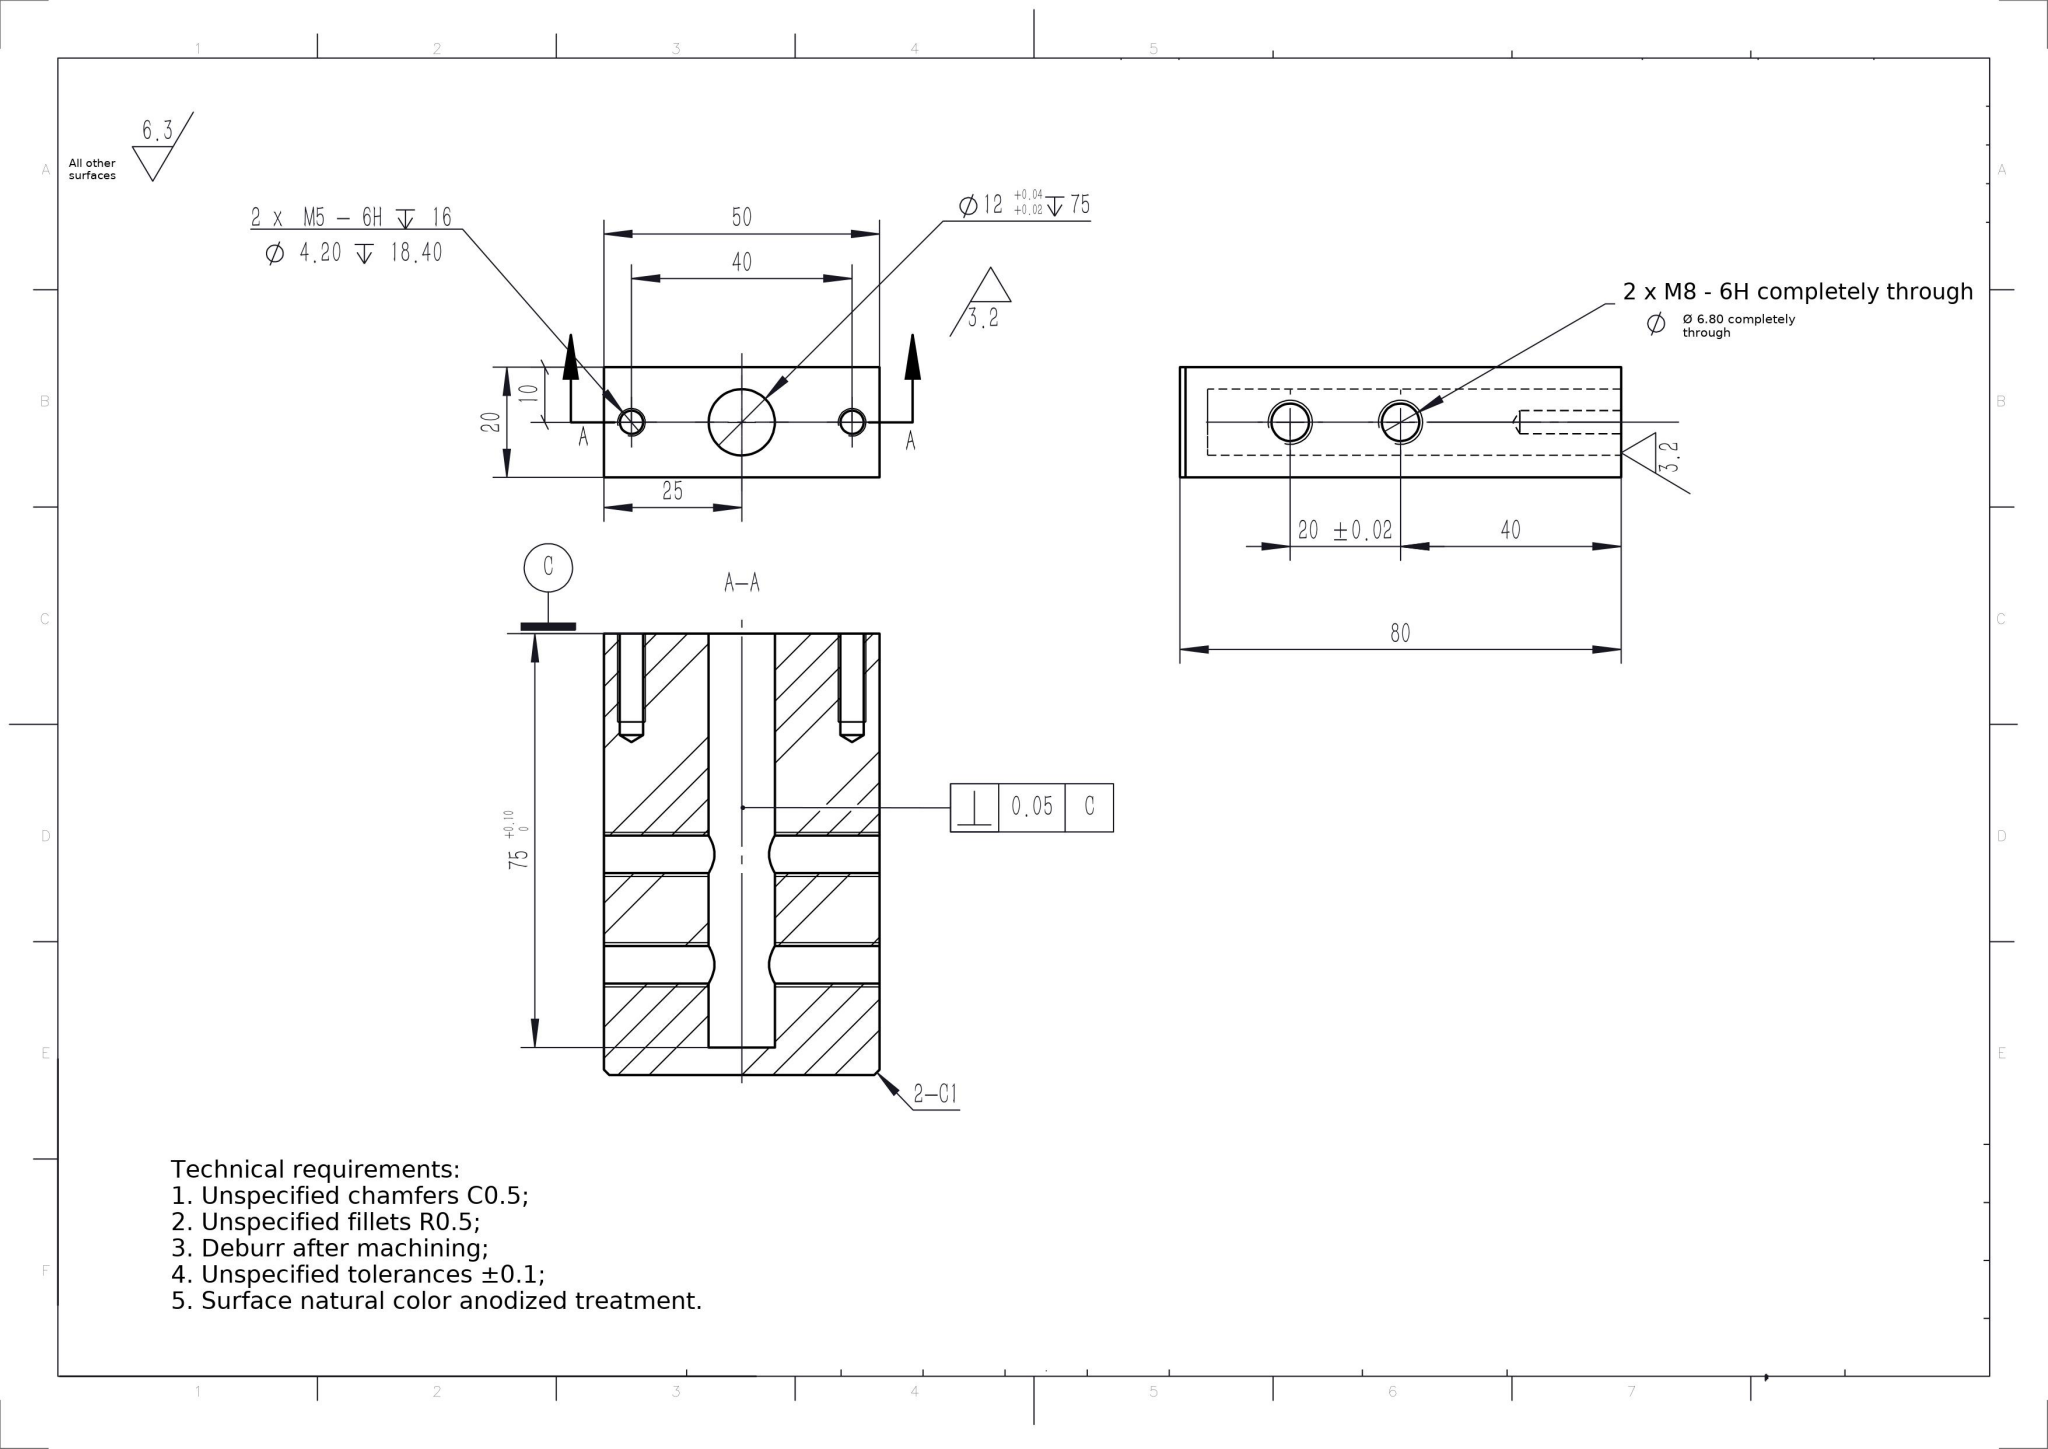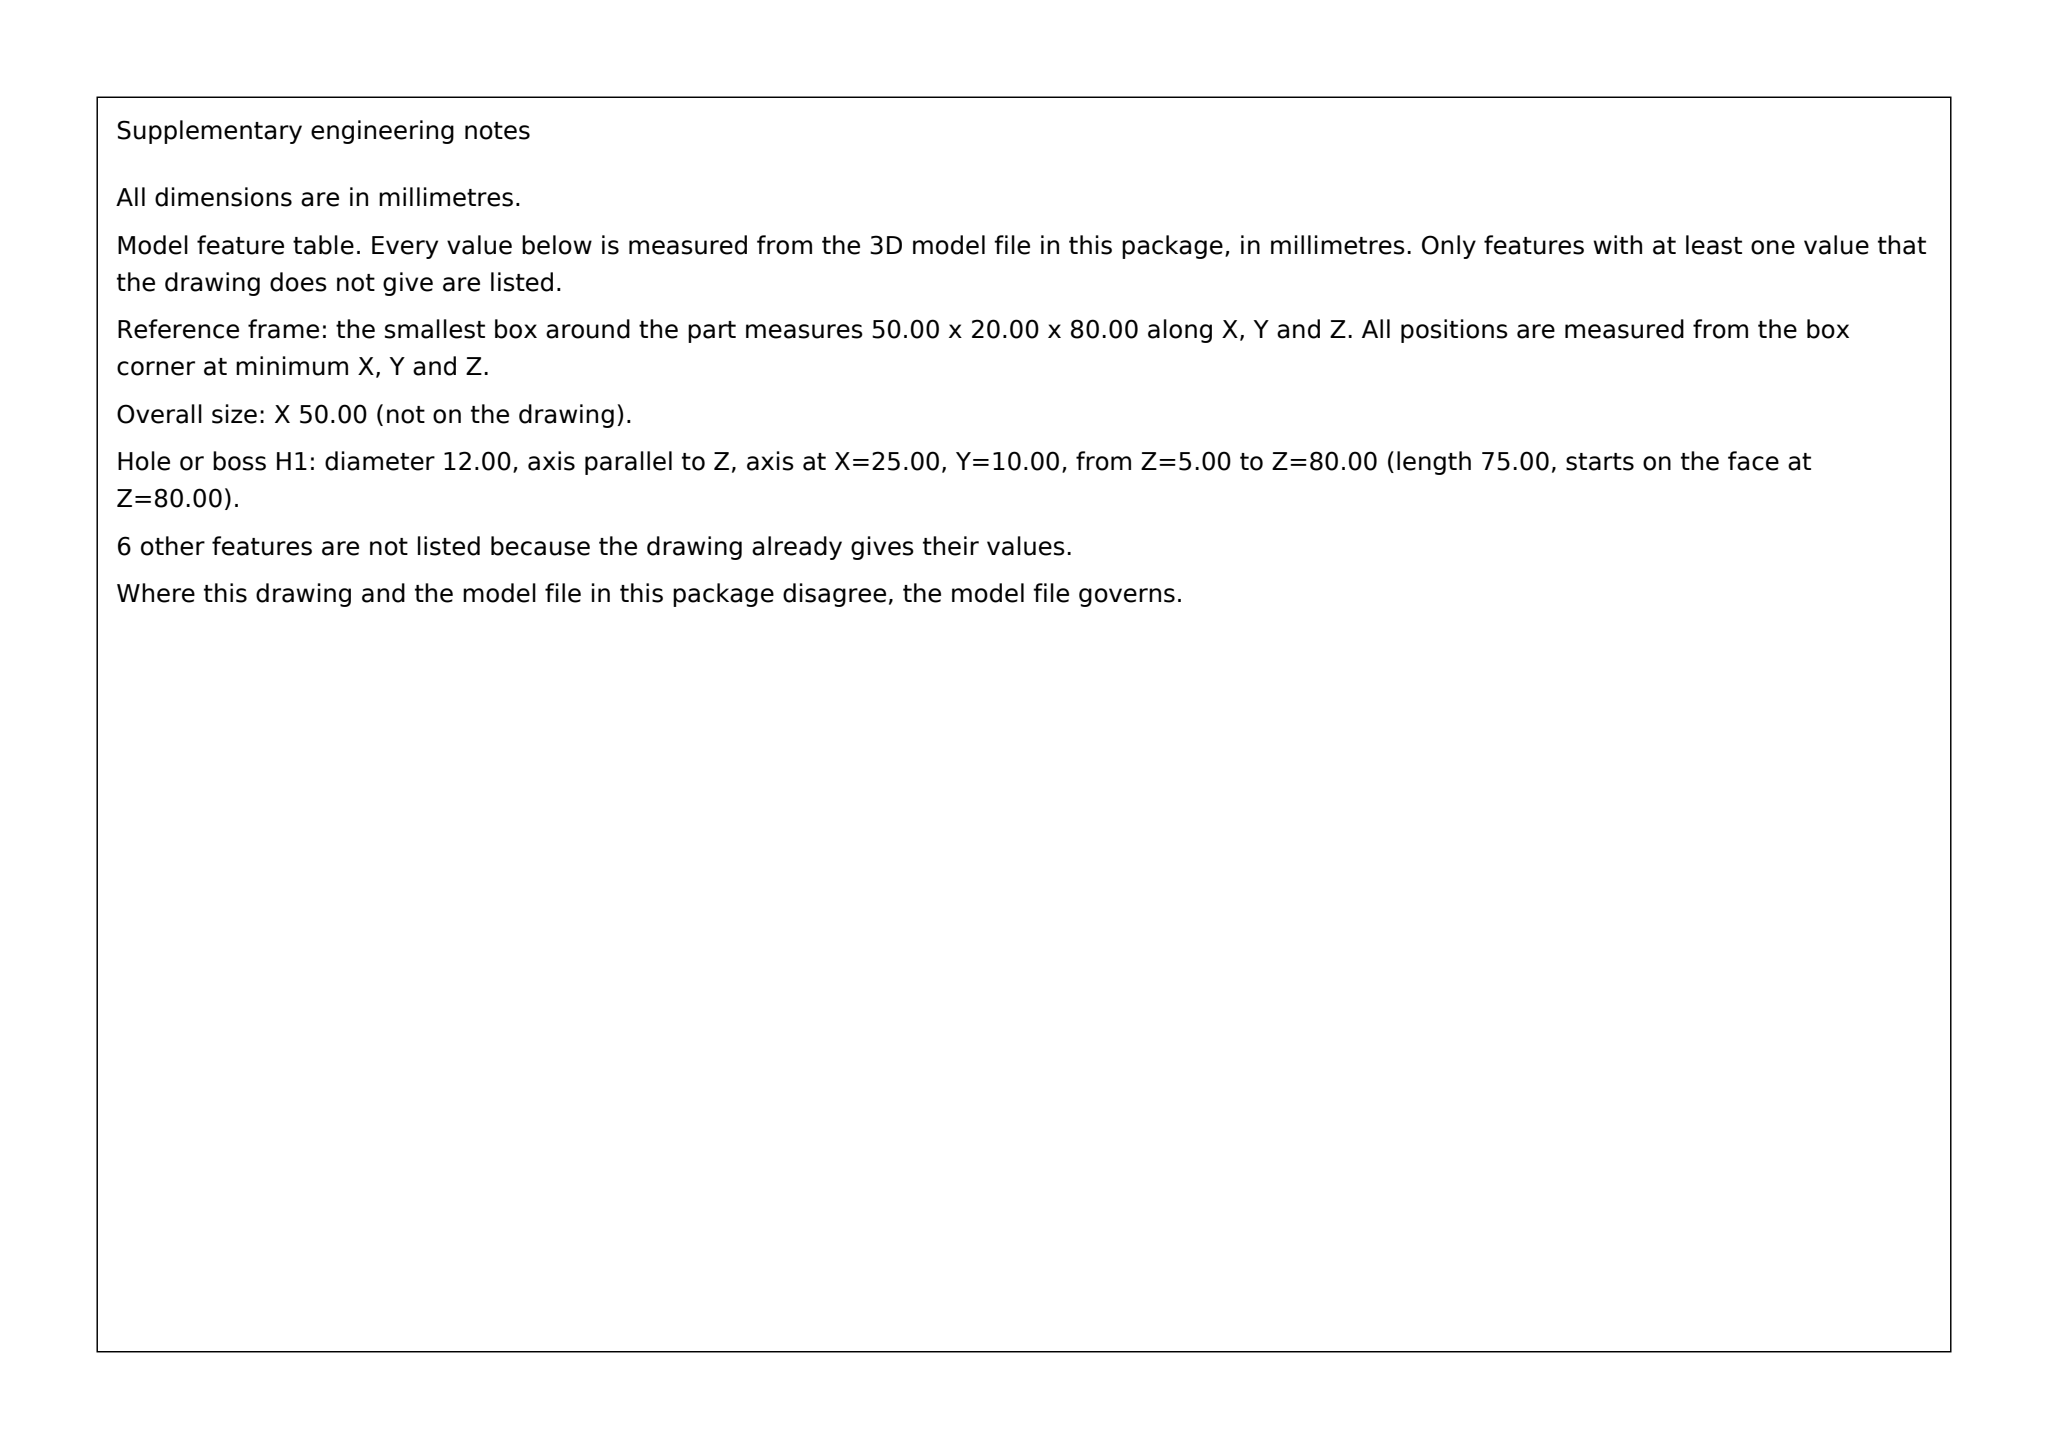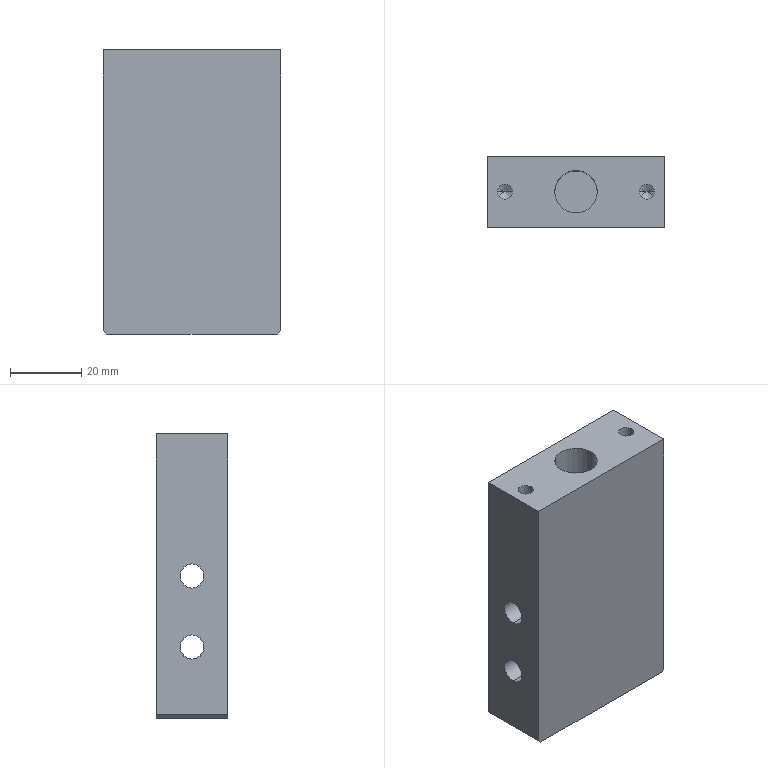Part | SolidWorks | mm | 1 solid | 27 faces | box 50 x 20 x 80 mm | volume 68180 mm3 | cylinder 14 | plane 9 | cone 4 | commonest cylinder face diameters 6.8 x8 4.2 x4 12 x2
build123d program:
from build123d import *

# Parameters (mm, degrees)
SKETCH1_W             = 50
SKETCH1_H             = 20
BOSS_EXTRUDE1_DEPTH   = 80
SKETCH2_R             = 6
CUT_EXTRUDE1_DEPTH    = 75
M8_TAPPED_HOLE1_D     = 6.8
M5_TAPPED_HOLE1_D     = 4.2
M5_TAPPED_HOLE1_DEPTH = 18.4
M5_TAPPED_HOLE1_TIP   = 1.262
CHAMFER1_SIZE         = 1


with BuildPart() as part:
    # Sketch1 → Boss-Extrude1 (new body)
    with BuildSketch(Plane.XY):
        Rectangle(SKETCH1_W, SKETCH1_H)
    extrude(amount=BOSS_EXTRUDE1_DEPTH)

    # Sketch2 → Cut-Extrude1 (cut)
    with BuildSketch(Plane.XY.offset(80)):
        Circle(SKETCH2_R)
    extrude(amount=-CUT_EXTRUDE1_DEPTH, mode=Mode.SUBTRACT)

    # M8 Tapped Hole1 (through all)
    with Locations(Plane(origin=(25, 0, 0), x_dir=(0, 0, -1), z_dir=(1, 0, 0))):
        with Locations((-40, 0), (-20, 0)):
            Hole(M8_TAPPED_HOLE1_D / 2)

    # M5 Tapped Hole1
    with Locations(Plane.XY.offset(80)):
        with Locations((-20, 0), (20, 0)):
            Hole(M5_TAPPED_HOLE1_D / 2, depth=M5_TAPPED_HOLE1_DEPTH)
            with Locations((0, 0, -(M5_TAPPED_HOLE1_DEPTH + M5_TAPPED_HOLE1_TIP / 2))):  # 118° drill point
                Cone(0, M5_TAPPED_HOLE1_D / 2, M5_TAPPED_HOLE1_TIP, mode=Mode.SUBTRACT)

    # Chamfer1
    chamfer1_edges = [part.edges().sort_by_distance(p)[0] for p in [
        (-25, 0, 0),
        (25, 0, 0),
    ]]
    chamfer(chamfer1_edges, length=CHAMFER1_SIZE)


solid = part.part